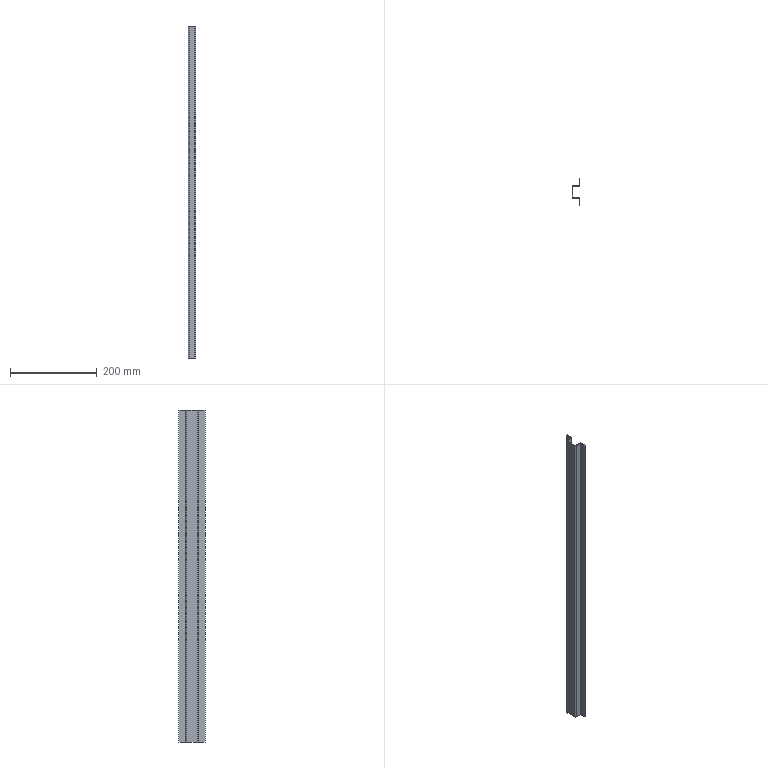Component | SolidWorks | UpperLeftSidePlate-1_UpperLeftOuterSidePanelStiffener-1 | 1 solid | 38 faces | box 18.4 x 60 x 766 mm | volume 104324 mm3 | plane 30 | cylinder 8 | commonest cylinder face diameters 5 x4 2 x4 | material 304
STEP:
#1=COLOUR_RGB('',0.7922,0.8196,0.9333);
#2=FILL_AREA_STYLE_COLOUR('',#1);
#3=FILL_AREA_STYLE('',(#2));
#4=SURFACE_STYLE_FILL_AREA(#3);
#5=SURFACE_SIDE_STYLE('',(#4));
#6=SURFACE_STYLE_USAGE(.BOTH.,#5);
#7=PRESENTATION_STYLE_ASSIGNMENT((#6));
#8=CARTESIAN_POINT('',(21.127,-3.735,78.388));
#9=VERTEX_POINT('',#8);
#10=CARTESIAN_POINT('',(21.127,-3.676,78.388));
#11=VERTEX_POINT('',#10);
#12=CARTESIAN_POINT('',(21.127,-3.735,78.388));
#13=DIRECTION('',(0.,1.,0.));
#14=VECTOR('',#13,39.37);
#15=LINE('',#12,#14);
#16=EDGE_CURVE('',#9,#11,#15,.T.);
#17=ORIENTED_EDGE('',*,*,#16,.F.);
#18=CARTESIAN_POINT('',(21.167,-3.775,78.388));
#19=VERTEX_POINT('',#18);
#20=CARTESIAN_POINT('',(21.127,-3.775,78.388));
#21=DIRECTION('',(-0.,0.,-1.));
#22=DIRECTION('',(-1.,0.,0.));
#23=AXIS2_PLACEMENT_3D('',#20,#21,#22);
#24=CIRCLE('',#23,0.03937);
#25=EDGE_CURVE('',#9,#19,#24,.T.);
#26=ORIENTED_EDGE('',*,*,#25,.T.);
#27=CARTESIAN_POINT('',(21.226,-3.775,78.388));
#28=VERTEX_POINT('',#27);
#29=CARTESIAN_POINT('',(21.226,-3.775,78.388));
#30=DIRECTION('',(-1.,0.,0.));
#31=VECTOR('',#30,39.37);
#32=LINE('',#29,#31);
#33=EDGE_CURVE('',#28,#19,#32,.T.);
#34=ORIENTED_EDGE('',*,*,#33,.F.);
#35=CARTESIAN_POINT('',(21.127,-3.775,78.388));
#36=DIRECTION('',(-0.,0.,-1.));
#37=DIRECTION('',(0.,1.,0.));
#38=AXIS2_PLACEMENT_3D('',#35,#36,#37);
#39=CIRCLE('',#38,0.09843);
#40=EDGE_CURVE('',#11,#28,#39,.T.);
#41=ORIENTED_EDGE('',*,*,#40,.F.);
#42=EDGE_LOOP('',(#17,#26,#34,#41));
#43=FACE_OUTER_BOUND('',#42,.T.);
#44=CARTESIAN_POINT('',(21.127,-3.735,78.388));
#45=DIRECTION('',(0.,-0.,1.));
#46=DIRECTION('',(1.,-0.,-0.));
#47=AXIS2_PLACEMENT_3D('',#44,#45,#46);
#48=PLANE('',#47);
#49=ADVANCED_FACE('',(#43),#48,.T.);
#50=CARTESIAN_POINT('',(20.6,-3.735,78.388));
#51=VERTEX_POINT('',#50);
#52=CARTESIAN_POINT('',(21.167,-3.735,78.388));
#53=DIRECTION('',(1.,-0.,-0.));
#54=VECTOR('',#53,39.37);
#55=LINE('',#52,#54);
#56=EDGE_CURVE('',#51,#9,#55,.T.);
#57=ORIENTED_EDGE('',*,*,#56,.T.);
#58=ORIENTED_EDGE('',*,*,#16,.T.);
#59=CARTESIAN_POINT('',(20.6,-3.676,78.388));
#60=VERTEX_POINT('',#59);
#61=CARTESIAN_POINT('',(21.167,-3.676,78.388));
#62=DIRECTION('',(1.,-0.,-0.));
#63=VECTOR('',#62,39.37);
#64=LINE('',#61,#63);
#65=EDGE_CURVE('',#60,#11,#64,.T.);
#66=ORIENTED_EDGE('',*,*,#65,.F.);
#67=CARTESIAN_POINT('',(20.6,-3.676,78.388));
#68=DIRECTION('',(-0.,-1.,-0.));
#69=VECTOR('',#68,39.37);
#70=LINE('',#67,#69);
#71=EDGE_CURVE('',#60,#51,#70,.T.);
#72=ORIENTED_EDGE('',*,*,#71,.T.);
#73=EDGE_LOOP('',(#57,#58,#66,#72));
#74=FACE_OUTER_BOUND('',#73,.T.);
#75=CARTESIAN_POINT('',(21.226,-3.775,78.388));
#76=DIRECTION('',(0.,-0.,1.));
#77=DIRECTION('',(1.,-0.,-0.));
#78=AXIS2_PLACEMENT_3D('',#75,#76,#77);
#79=PLANE('',#78);
#80=ADVANCED_FACE('',(#74),#79,.T.);
#81=CARTESIAN_POINT('',(21.167,-3.775,48.23));
#82=VERTEX_POINT('',#81);
#83=CARTESIAN_POINT('',(21.226,-3.775,48.23));
#84=VERTEX_POINT('',#83);
#85=CARTESIAN_POINT('',(21.167,-3.775,48.23));
#86=DIRECTION('',(1.,-0.,-0.));
#87=VECTOR('',#86,39.37);
#88=LINE('',#85,#87);
#89=EDGE_CURVE('',#82,#84,#88,.T.);
#90=ORIENTED_EDGE('',*,*,#89,.F.);
#91=CARTESIAN_POINT('',(21.127,-3.735,48.23));
#92=VERTEX_POINT('',#91);
#93=CARTESIAN_POINT('',(21.127,-3.775,48.23));
#94=DIRECTION('',(-0.,0.,-1.));
#95=DIRECTION('',(-1.,0.,0.));
#96=AXIS2_PLACEMENT_3D('',#93,#94,#95);
#97=CIRCLE('',#96,0.03937);
#98=EDGE_CURVE('',#92,#82,#97,.T.);
#99=ORIENTED_EDGE('',*,*,#98,.F.);
#100=CARTESIAN_POINT('',(21.127,-3.676,48.23));
#101=VERTEX_POINT('',#100);
#102=CARTESIAN_POINT('',(21.127,-3.676,48.23));
#103=DIRECTION('',(-0.,-1.,-0.));
#104=VECTOR('',#103,39.37);
#105=LINE('',#102,#104);
#106=EDGE_CURVE('',#101,#92,#105,.T.);
#107=ORIENTED_EDGE('',*,*,#106,.F.);
#108=CARTESIAN_POINT('',(21.127,-3.775,48.23));
#109=DIRECTION('',(-0.,0.,-1.));
#110=DIRECTION('',(0.,1.,0.));
#111=AXIS2_PLACEMENT_3D('',#108,#109,#110);
#112=CIRCLE('',#111,0.09843);
#113=EDGE_CURVE('',#101,#84,#112,.T.);
#114=ORIENTED_EDGE('',*,*,#113,.T.);
#115=EDGE_LOOP('',(#90,#99,#107,#114));
#116=FACE_OUTER_BOUND('',#115,.T.);
#117=CARTESIAN_POINT('',(21.167,-3.775,48.23));
#118=DIRECTION('',(-0.,0.,-1.));
#119=DIRECTION('',(-1.,0.,0.));
#120=AXIS2_PLACEMENT_3D('',#117,#118,#119);
#121=PLANE('',#120);
#122=ADVANCED_FACE('',(#116),#121,.T.);
#123=CARTESIAN_POINT('',(21.167,-4.326,48.23));
#124=VERTEX_POINT('',#123);
#125=CARTESIAN_POINT('',(21.167,-4.326,48.23));
#126=DIRECTION('',(-0.,-1.,-0.));
#127=VECTOR('',#126,39.37);
#128=LINE('',#125,#127);
#129=EDGE_CURVE('',#82,#124,#128,.T.);
#130=ORIENTED_EDGE('',*,*,#129,.F.);
#131=ORIENTED_EDGE('',*,*,#89,.T.);
#132=CARTESIAN_POINT('',(21.226,-4.326,48.23));
#133=VERTEX_POINT('',#132);
#134=CARTESIAN_POINT('',(21.226,-4.326,48.23));
#135=DIRECTION('',(-0.,-1.,-0.));
#136=VECTOR('',#135,39.37);
#137=LINE('',#134,#136);
#138=EDGE_CURVE('',#84,#133,#137,.T.);
#139=ORIENTED_EDGE('',*,*,#138,.T.);
#140=CARTESIAN_POINT('',(21.226,-4.326,48.23));
#141=DIRECTION('',(-1.,0.,0.));
#142=VECTOR('',#141,39.37);
#143=LINE('',#140,#142);
#144=EDGE_CURVE('',#133,#124,#143,.T.);
#145=ORIENTED_EDGE('',*,*,#144,.T.);
#146=EDGE_LOOP('',(#130,#131,#139,#145));
#147=FACE_OUTER_BOUND('',#146,.T.);
#148=CARTESIAN_POINT('',(21.127,-3.676,48.23));
#149=DIRECTION('',(-0.,0.,-1.));
#150=DIRECTION('',(-1.,0.,0.));
#151=AXIS2_PLACEMENT_3D('',#148,#149,#150);
#152=PLANE('',#151);
#153=ADVANCED_FACE('',(#147),#152,.T.);
#154=CARTESIAN_POINT('',(20.501,-3.637,78.388));
#155=VERTEX_POINT('',#154);
#156=CARTESIAN_POINT('',(20.56,-3.637,78.388));
#157=VERTEX_POINT('',#156);
#158=CARTESIAN_POINT('',(20.501,-3.637,78.388));
#159=DIRECTION('',(1.,-0.,-0.));
#160=VECTOR('',#159,39.37);
#161=LINE('',#158,#160);
#162=EDGE_CURVE('',#155,#157,#161,.T.);
#163=ORIENTED_EDGE('',*,*,#162,.F.);
#164=CARTESIAN_POINT('',(20.6,-3.637,78.388));
#165=DIRECTION('',(0.,-0.,1.));
#166=DIRECTION('',(1.,-0.,0.));
#167=AXIS2_PLACEMENT_3D('',#164,#165,#166);
#168=CIRCLE('',#167,0.09843);
#169=EDGE_CURVE('',#155,#51,#168,.T.);
#170=ORIENTED_EDGE('',*,*,#169,.T.);
#171=ORIENTED_EDGE('',*,*,#71,.F.);
#172=CARTESIAN_POINT('',(20.6,-3.637,78.388));
#173=DIRECTION('',(0.,-0.,1.));
#174=DIRECTION('',(0.,1.,0.));
#175=AXIS2_PLACEMENT_3D('',#172,#173,#174);
#176=CIRCLE('',#175,0.03937);
#177=EDGE_CURVE('',#157,#60,#176,.T.);
#178=ORIENTED_EDGE('',*,*,#177,.F.);
#179=EDGE_LOOP('',(#163,#170,#171,#178));
#180=FACE_OUTER_BOUND('',#179,.T.);
#181=CARTESIAN_POINT('',(20.501,-3.637,78.388));
#182=DIRECTION('',(0.,-0.,1.));
#183=DIRECTION('',(1.,-0.,-0.));
#184=AXIS2_PLACEMENT_3D('',#181,#182,#183);
#185=PLANE('',#184);
#186=ADVANCED_FACE('',(#180),#185,.T.);
#187=CARTESIAN_POINT('',(20.501,-2.653,78.388));
#188=VERTEX_POINT('',#187);
#189=CARTESIAN_POINT('',(20.501,-3.735,78.388));
#190=DIRECTION('',(-0.,-1.,-0.));
#191=VECTOR('',#190,39.37);
#192=LINE('',#189,#191);
#193=EDGE_CURVE('',#188,#155,#192,.T.);
#194=ORIENTED_EDGE('',*,*,#193,.T.);
#195=ORIENTED_EDGE('',*,*,#162,.T.);
#196=CARTESIAN_POINT('',(20.56,-2.653,78.388));
#197=VERTEX_POINT('',#196);
#198=CARTESIAN_POINT('',(20.56,-3.735,78.388));
#199=DIRECTION('',(-0.,-1.,-0.));
#200=VECTOR('',#199,39.37);
#201=LINE('',#198,#200);
#202=EDGE_CURVE('',#197,#157,#201,.T.);
#203=ORIENTED_EDGE('',*,*,#202,.F.);
#204=CARTESIAN_POINT('',(20.56,-2.653,78.388));
#205=DIRECTION('',(-1.,0.,0.));
#206=VECTOR('',#205,39.37);
#207=LINE('',#204,#206);
#208=EDGE_CURVE('',#197,#188,#207,.T.);
#209=ORIENTED_EDGE('',*,*,#208,.T.);
#210=EDGE_LOOP('',(#194,#195,#203,#209));
#211=FACE_OUTER_BOUND('',#210,.T.);
#212=CARTESIAN_POINT('',(20.6,-3.676,78.388));
#213=DIRECTION('',(0.,-0.,1.));
#214=DIRECTION('',(1.,-0.,-0.));
#215=AXIS2_PLACEMENT_3D('',#212,#213,#214);
#216=PLANE('',#215);
#217=ADVANCED_FACE('',(#211),#216,.T.);
#218=CARTESIAN_POINT('',(20.6,-3.735,48.23));
#219=VERTEX_POINT('',#218);
#220=CARTESIAN_POINT('',(20.6,-3.676,48.23));
#221=VERTEX_POINT('',#220);
#222=CARTESIAN_POINT('',(20.6,-3.735,48.23));
#223=DIRECTION('',(0.,1.,0.));
#224=VECTOR('',#223,39.37);
#225=LINE('',#222,#224);
#226=EDGE_CURVE('',#219,#221,#225,.T.);
#227=ORIENTED_EDGE('',*,*,#226,.F.);
#228=CARTESIAN_POINT('',(20.501,-3.637,48.23));
#229=VERTEX_POINT('',#228);
#230=CARTESIAN_POINT('',(20.6,-3.637,48.23));
#231=DIRECTION('',(0.,-0.,1.));
#232=DIRECTION('',(1.,-0.,0.));
#233=AXIS2_PLACEMENT_3D('',#230,#231,#232);
#234=CIRCLE('',#233,0.09843);
#235=EDGE_CURVE('',#229,#219,#234,.T.);
#236=ORIENTED_EDGE('',*,*,#235,.F.);
#237=CARTESIAN_POINT('',(20.56,-3.637,48.23));
#238=VERTEX_POINT('',#237);
#239=CARTESIAN_POINT('',(20.56,-3.637,48.23));
#240=DIRECTION('',(-1.,0.,0.));
#241=VECTOR('',#240,39.37);
#242=LINE('',#239,#241);
#243=EDGE_CURVE('',#238,#229,#242,.T.);
#244=ORIENTED_EDGE('',*,*,#243,.F.);
#245=CARTESIAN_POINT('',(20.6,-3.637,48.23));
#246=DIRECTION('',(0.,-0.,1.));
#247=DIRECTION('',(0.,1.,0.));
#248=AXIS2_PLACEMENT_3D('',#245,#246,#247);
#249=CIRCLE('',#248,0.03937);
#250=EDGE_CURVE('',#238,#221,#249,.T.);
#251=ORIENTED_EDGE('',*,*,#250,.T.);
#252=EDGE_LOOP('',(#227,#236,#244,#251));
#253=FACE_OUTER_BOUND('',#252,.T.);
#254=CARTESIAN_POINT('',(20.6,-3.735,48.23));
#255=DIRECTION('',(-0.,0.,-1.));
#256=DIRECTION('',(-1.,0.,0.));
#257=AXIS2_PLACEMENT_3D('',#254,#255,#256);
#258=PLANE('',#257);
#259=ADVANCED_FACE('',(#253),#258,.T.);
#260=CARTESIAN_POINT('',(21.167,-3.735,48.23));
#261=DIRECTION('',(1.,-0.,-0.));
#262=VECTOR('',#261,39.37);
#263=LINE('',#260,#262);
#264=EDGE_CURVE('',#219,#92,#263,.T.);
#265=ORIENTED_EDGE('',*,*,#264,.F.);
#266=ORIENTED_EDGE('',*,*,#226,.T.);
#267=CARTESIAN_POINT('',(21.167,-3.676,48.23));
#268=DIRECTION('',(1.,-0.,-0.));
#269=VECTOR('',#268,39.37);
#270=LINE('',#267,#269);
#271=EDGE_CURVE('',#221,#101,#270,.T.);
#272=ORIENTED_EDGE('',*,*,#271,.T.);
#273=ORIENTED_EDGE('',*,*,#106,.T.);
#274=EDGE_LOOP('',(#265,#266,#272,#273));
#275=FACE_OUTER_BOUND('',#274,.T.);
#276=CARTESIAN_POINT('',(20.56,-3.637,48.23));
#277=DIRECTION('',(-0.,0.,-1.));
#278=DIRECTION('',(-1.,0.,0.));
#279=AXIS2_PLACEMENT_3D('',#276,#277,#278);
#280=PLANE('',#279);
#281=ADVANCED_FACE('',(#275),#280,.T.);
#282=CARTESIAN_POINT('',(20.6,-2.554,78.388));
#283=VERTEX_POINT('',#282);
#284=CARTESIAN_POINT('',(20.6,-2.613,78.388));
#285=VERTEX_POINT('',#284);
#286=CARTESIAN_POINT('',(20.6,-2.554,78.388));
#287=DIRECTION('',(-0.,-1.,-0.));
#288=VECTOR('',#287,39.37);
#289=LINE('',#286,#288);
#290=EDGE_CURVE('',#283,#285,#289,.T.);
#291=ORIENTED_EDGE('',*,*,#290,.F.);
#292=CARTESIAN_POINT('',(20.6,-2.653,78.388));
#293=DIRECTION('',(0.,-0.,1.));
#294=DIRECTION('',(1.,-0.,0.));
#295=AXIS2_PLACEMENT_3D('',#292,#293,#294);
#296=CIRCLE('',#295,0.09843);
#297=EDGE_CURVE('',#283,#188,#296,.T.);
#298=ORIENTED_EDGE('',*,*,#297,.T.);
#299=ORIENTED_EDGE('',*,*,#208,.F.);
#300=CARTESIAN_POINT('',(20.6,-2.653,78.388));
#301=DIRECTION('',(0.,-0.,1.));
#302=DIRECTION('',(0.,1.,0.));
#303=AXIS2_PLACEMENT_3D('',#300,#301,#302);
#304=CIRCLE('',#303,0.03937);
#305=EDGE_CURVE('',#285,#197,#304,.T.);
#306=ORIENTED_EDGE('',*,*,#305,.F.);
#307=EDGE_LOOP('',(#291,#298,#299,#306));
#308=FACE_OUTER_BOUND('',#307,.T.);
#309=CARTESIAN_POINT('',(20.6,-2.554,78.388));
#310=DIRECTION('',(0.,-0.,1.));
#311=DIRECTION('',(1.,-0.,-0.));
#312=AXIS2_PLACEMENT_3D('',#309,#310,#311);
#313=PLANE('',#312);
#314=ADVANCED_FACE('',(#308),#313,.T.);
#315=CARTESIAN_POINT('',(21.127,-2.554,78.388));
#316=VERTEX_POINT('',#315);
#317=CARTESIAN_POINT('',(21.167,-2.554,78.388));
#318=DIRECTION('',(-1.,0.,0.));
#319=VECTOR('',#318,39.37);
#320=LINE('',#317,#319);
#321=EDGE_CURVE('',#316,#283,#320,.T.);
#322=ORIENTED_EDGE('',*,*,#321,.T.);
#323=ORIENTED_EDGE('',*,*,#290,.T.);
#324=CARTESIAN_POINT('',(21.127,-2.613,78.388));
#325=VERTEX_POINT('',#324);
#326=CARTESIAN_POINT('',(21.167,-2.613,78.388));
#327=DIRECTION('',(-1.,0.,0.));
#328=VECTOR('',#327,39.37);
#329=LINE('',#326,#328);
#330=EDGE_CURVE('',#325,#285,#329,.T.);
#331=ORIENTED_EDGE('',*,*,#330,.F.);
#332=CARTESIAN_POINT('',(21.127,-2.613,78.388));
#333=DIRECTION('',(0.,1.,0.));
#334=VECTOR('',#333,39.37);
#335=LINE('',#332,#334);
#336=EDGE_CURVE('',#325,#316,#335,.T.);
#337=ORIENTED_EDGE('',*,*,#336,.T.);
#338=EDGE_LOOP('',(#322,#323,#331,#337));
#339=FACE_OUTER_BOUND('',#338,.T.);
#340=CARTESIAN_POINT('',(20.56,-2.653,78.388));
#341=DIRECTION('',(0.,-0.,1.));
#342=DIRECTION('',(1.,-0.,-0.));
#343=AXIS2_PLACEMENT_3D('',#340,#341,#342);
#344=PLANE('',#343);
#345=ADVANCED_FACE('',(#339),#344,.T.);
#346=CARTESIAN_POINT('',(20.501,-2.653,48.23));
#347=VERTEX_POINT('',#346);
#348=CARTESIAN_POINT('',(20.56,-2.653,48.23));
#349=VERTEX_POINT('',#348);
#350=CARTESIAN_POINT('',(20.501,-2.653,48.23));
#351=DIRECTION('',(1.,-0.,-0.));
#352=VECTOR('',#351,39.37);
#353=LINE('',#350,#352);
#354=EDGE_CURVE('',#347,#349,#353,.T.);
#355=ORIENTED_EDGE('',*,*,#354,.F.);
#356=CARTESIAN_POINT('',(20.6,-2.554,48.23));
#357=VERTEX_POINT('',#356);
#358=CARTESIAN_POINT('',(20.6,-2.653,48.23));
#359=DIRECTION('',(0.,-0.,1.));
#360=DIRECTION('',(1.,-0.,0.));
#361=AXIS2_PLACEMENT_3D('',#358,#359,#360);
#362=CIRCLE('',#361,0.09843);
#363=EDGE_CURVE('',#357,#347,#362,.T.);
#364=ORIENTED_EDGE('',*,*,#363,.F.);
#365=CARTESIAN_POINT('',(20.6,-2.613,48.23));
#366=VERTEX_POINT('',#365);
#367=CARTESIAN_POINT('',(20.6,-2.613,48.23));
#368=DIRECTION('',(0.,1.,0.));
#369=VECTOR('',#368,39.37);
#370=LINE('',#367,#369);
#371=EDGE_CURVE('',#366,#357,#370,.T.);
#372=ORIENTED_EDGE('',*,*,#371,.F.);
#373=CARTESIAN_POINT('',(20.6,-2.653,48.23));
#374=DIRECTION('',(0.,-0.,1.));
#375=DIRECTION('',(0.,1.,0.));
#376=AXIS2_PLACEMENT_3D('',#373,#374,#375);
#377=CIRCLE('',#376,0.03937);
#378=EDGE_CURVE('',#366,#349,#377,.T.);
#379=ORIENTED_EDGE('',*,*,#378,.T.);
#380=EDGE_LOOP('',(#355,#364,#372,#379));
#381=FACE_OUTER_BOUND('',#380,.T.);
#382=CARTESIAN_POINT('',(20.501,-2.653,48.23));
#383=DIRECTION('',(-0.,0.,-1.));
#384=DIRECTION('',(-1.,0.,0.));
#385=AXIS2_PLACEMENT_3D('',#382,#383,#384);
#386=PLANE('',#385);
#387=ADVANCED_FACE('',(#381),#386,.T.);
#388=CARTESIAN_POINT('',(20.501,-3.735,48.23));
#389=DIRECTION('',(-0.,-1.,-0.));
#390=VECTOR('',#389,39.37);
#391=LINE('',#388,#390);
#392=EDGE_CURVE('',#347,#229,#391,.T.);
#393=ORIENTED_EDGE('',*,*,#392,.F.);
#394=ORIENTED_EDGE('',*,*,#354,.T.);
#395=CARTESIAN_POINT('',(20.56,-3.735,48.23));
#396=DIRECTION('',(-0.,-1.,-0.));
#397=VECTOR('',#396,39.37);
#398=LINE('',#395,#397);
#399=EDGE_CURVE('',#349,#238,#398,.T.);
#400=ORIENTED_EDGE('',*,*,#399,.T.);
#401=ORIENTED_EDGE('',*,*,#243,.T.);
#402=EDGE_LOOP('',(#393,#394,#400,#401));
#403=FACE_OUTER_BOUND('',#402,.T.);
#404=CARTESIAN_POINT('',(20.6,-2.613,48.23));
#405=DIRECTION('',(-0.,0.,-1.));
#406=DIRECTION('',(-1.,0.,0.));
#407=AXIS2_PLACEMENT_3D('',#404,#405,#406);
#408=PLANE('',#407);
#409=ADVANCED_FACE('',(#403),#408,.T.);
#410=CARTESIAN_POINT('',(21.167,-2.515,78.388));
#411=VERTEX_POINT('',#410);
#412=CARTESIAN_POINT('',(21.226,-2.515,78.388));
#413=VERTEX_POINT('',#412);
#414=CARTESIAN_POINT('',(21.167,-2.515,78.388));
#415=DIRECTION('',(1.,0.,-0.));
#416=VECTOR('',#415,39.37);
#417=LINE('',#414,#416);
#418=EDGE_CURVE('',#411,#413,#417,.T.);
#419=ORIENTED_EDGE('',*,*,#418,.F.);
#420=CARTESIAN_POINT('',(21.127,-2.515,78.388));
#421=DIRECTION('',(-0.,0.,-1.));
#422=DIRECTION('',(-1.,0.,0.));
#423=AXIS2_PLACEMENT_3D('',#420,#421,#422);
#424=CIRCLE('',#423,0.03937);
#425=EDGE_CURVE('',#411,#316,#424,.T.);
#426=ORIENTED_EDGE('',*,*,#425,.T.);
#427=ORIENTED_EDGE('',*,*,#336,.F.);
#428=CARTESIAN_POINT('',(21.127,-2.515,78.388));
#429=DIRECTION('',(-0.,0.,-1.));
#430=DIRECTION('',(0.,1.,0.));
#431=AXIS2_PLACEMENT_3D('',#428,#429,#430);
#432=CIRCLE('',#431,0.09843);
#433=EDGE_CURVE('',#413,#325,#432,.T.);
#434=ORIENTED_EDGE('',*,*,#433,.F.);
#435=EDGE_LOOP('',(#419,#426,#427,#434));
#436=FACE_OUTER_BOUND('',#435,.T.);
#437=CARTESIAN_POINT('',(21.167,-2.515,78.388));
#438=DIRECTION('',(0.,-0.,1.));
#439=DIRECTION('',(1.,-0.,-0.));
#440=AXIS2_PLACEMENT_3D('',#437,#438,#439);
#441=PLANE('',#440);
#442=ADVANCED_FACE('',(#436),#441,.T.);
#443=CARTESIAN_POINT('',(21.167,-1.964,78.388));
#444=VERTEX_POINT('',#443);
#445=CARTESIAN_POINT('',(21.167,-1.964,78.388));
#446=DIRECTION('',(-0.,-1.,-0.));
#447=VECTOR('',#446,39.37);
#448=LINE('',#445,#447);
#449=EDGE_CURVE('',#444,#411,#448,.T.);
#450=ORIENTED_EDGE('',*,*,#449,.T.);
#451=ORIENTED_EDGE('',*,*,#418,.T.);
#452=CARTESIAN_POINT('',(21.226,-1.964,78.388));
#453=VERTEX_POINT('',#452);
#454=CARTESIAN_POINT('',(21.226,-1.964,78.388));
#455=DIRECTION('',(-0.,-1.,-0.));
#456=VECTOR('',#455,39.37);
#457=LINE('',#454,#456);
#458=EDGE_CURVE('',#453,#413,#457,.T.);
#459=ORIENTED_EDGE('',*,*,#458,.F.);
#460=CARTESIAN_POINT('',(21.167,-1.964,78.388));
#461=DIRECTION('',(1.,-0.,-0.));
#462=VECTOR('',#461,39.37);
#463=LINE('',#460,#462);
#464=EDGE_CURVE('',#444,#453,#463,.T.);
#465=ORIENTED_EDGE('',*,*,#464,.F.);
#466=EDGE_LOOP('',(#450,#451,#459,#465));
#467=FACE_OUTER_BOUND('',#466,.T.);
#468=CARTESIAN_POINT('',(21.127,-2.613,78.388));
#469=DIRECTION('',(0.,-0.,1.));
#470=DIRECTION('',(1.,-0.,-0.));
#471=AXIS2_PLACEMENT_3D('',#468,#469,#470);
#472=PLANE('',#471);
#473=ADVANCED_FACE('',(#467),#472,.T.);
#474=CARTESIAN_POINT('',(21.127,-2.554,48.23));
#475=VERTEX_POINT('',#474);
#476=CARTESIAN_POINT('',(21.127,-2.613,48.23));
#477=VERTEX_POINT('',#476);
#478=CARTESIAN_POINT('',(21.127,-2.554,48.23));
#479=DIRECTION('',(-0.,-1.,-0.));
#480=VECTOR('',#479,39.37);
#481=LINE('',#478,#480);
#482=EDGE_CURVE('',#475,#477,#481,.T.);
#483=ORIENTED_EDGE('',*,*,#482,.F.);
#484=CARTESIAN_POINT('',(21.167,-2.515,48.23));
#485=VERTEX_POINT('',#484);
#486=CARTESIAN_POINT('',(21.127,-2.515,48.23));
#487=DIRECTION('',(-0.,0.,-1.));
#488=DIRECTION('',(-1.,0.,0.));
#489=AXIS2_PLACEMENT_3D('',#486,#487,#488);
#490=CIRCLE('',#489,0.03937);
#491=EDGE_CURVE('',#485,#475,#490,.T.);
#492=ORIENTED_EDGE('',*,*,#491,.F.);
#493=CARTESIAN_POINT('',(21.226,-2.515,48.23));
#494=VERTEX_POINT('',#493);
#495=CARTESIAN_POINT('',(21.226,-2.515,48.23));
#496=DIRECTION('',(-1.,-0.,0.));
#497=VECTOR('',#496,39.37);
#498=LINE('',#495,#497);
#499=EDGE_CURVE('',#494,#485,#498,.T.);
#500=ORIENTED_EDGE('',*,*,#499,.F.);
#501=CARTESIAN_POINT('',(21.127,-2.515,48.23));
#502=DIRECTION('',(-0.,0.,-1.));
#503=DIRECTION('',(0.,1.,0.));
#504=AXIS2_PLACEMENT_3D('',#501,#502,#503);
#505=CIRCLE('',#504,0.09843);
#506=EDGE_CURVE('',#494,#477,#505,.T.);
#507=ORIENTED_EDGE('',*,*,#506,.T.);
#508=EDGE_LOOP('',(#483,#492,#500,#507));
#509=FACE_OUTER_BOUND('',#508,.T.);
#510=CARTESIAN_POINT('',(21.127,-2.554,48.23));
#511=DIRECTION('',(-0.,0.,-1.));
#512=DIRECTION('',(-1.,0.,0.));
#513=AXIS2_PLACEMENT_3D('',#510,#511,#512);
#514=PLANE('',#513);
#515=ADVANCED_FACE('',(#509),#514,.T.);
#516=CARTESIAN_POINT('',(21.167,-2.554,48.23));
#517=DIRECTION('',(-1.,0.,0.));
#518=VECTOR('',#517,39.37);
#519=LINE('',#516,#518);
#520=EDGE_CURVE('',#475,#357,#519,.T.);
#521=ORIENTED_EDGE('',*,*,#520,.F.);
#522=ORIENTED_EDGE('',*,*,#482,.T.);
#523=CARTESIAN_POINT('',(21.167,-2.613,48.23));
#524=DIRECTION('',(-1.,0.,0.));
#525=VECTOR('',#524,39.37);
#526=LINE('',#523,#525);
#527=EDGE_CURVE('',#477,#366,#526,.T.);
#528=ORIENTED_EDGE('',*,*,#527,.T.);
#529=ORIENTED_EDGE('',*,*,#371,.T.);
#530=EDGE_LOOP('',(#521,#522,#528,#529));
#531=FACE_OUTER_BOUND('',#530,.T.);
#532=CARTESIAN_POINT('',(21.226,-2.515,48.23));
#533=DIRECTION('',(-0.,0.,-1.));
#534=DIRECTION('',(-1.,0.,0.));
#535=AXIS2_PLACEMENT_3D('',#532,#533,#534);
#536=PLANE('',#535);
#537=ADVANCED_FACE('',(#531),#536,.T.);
#538=ORIENTED_EDGE('',*,*,#129,.T.);
#539=CARTESIAN_POINT('',(21.167,-4.326,78.388));
#540=VERTEX_POINT('',#539);
#541=CARTESIAN_POINT('',(21.167,-4.326,78.388));
#542=DIRECTION('',(-0.,0.,-1.));
#543=VECTOR('',#542,39.37);
#544=LINE('',#541,#543);
#545=EDGE_CURVE('',#540,#124,#544,.T.);
#546=ORIENTED_EDGE('',*,*,#545,.F.);
#547=CARTESIAN_POINT('',(21.167,-4.326,78.388));
#548=DIRECTION('',(-0.,-1.,-0.));
#549=VECTOR('',#548,39.37);
#550=LINE('',#547,#549);
#551=EDGE_CURVE('',#19,#540,#550,.T.);
#552=ORIENTED_EDGE('',*,*,#551,.F.);
#553=CARTESIAN_POINT('',(21.167,-3.775,78.388));
#554=DIRECTION('',(-0.,0.,-1.));
#555=VECTOR('',#554,39.37);
#556=LINE('',#553,#555);
#557=EDGE_CURVE('',#19,#82,#556,.T.);
#558=ORIENTED_EDGE('',*,*,#557,.T.);
#559=EDGE_LOOP('',(#538,#546,#552,#558));
#560=FACE_OUTER_BOUND('',#559,.T.);
#561=CARTESIAN_POINT('',(21.167,-4.326,78.388));
#562=DIRECTION('',(1.,-0.,-0.));
#563=DIRECTION('',(0.,1.,0.));
#564=AXIS2_PLACEMENT_3D('',#561,#562,#563);
#565=PLANE('',#564);
#566=ADVANCED_FACE('',(#560),#565,.F.);
#567=ORIENTED_EDGE('',*,*,#144,.F.);
#568=CARTESIAN_POINT('',(21.226,-4.326,78.388));
#569=VERTEX_POINT('',#568);
#570=CARTESIAN_POINT('',(21.226,-4.326,78.388));
#571=DIRECTION('',(-0.,0.,-1.));
#572=VECTOR('',#571,39.37);
#573=LINE('',#570,#572);
#574=EDGE_CURVE('',#569,#133,#573,.T.);
#575=ORIENTED_EDGE('',*,*,#574,.F.);
#576=CARTESIAN_POINT('',(21.226,-4.326,78.388));
#577=DIRECTION('',(-1.,0.,0.));
#578=VECTOR('',#577,39.37);
#579=LINE('',#576,#578);
#580=EDGE_CURVE('',#569,#540,#579,.T.);
#581=ORIENTED_EDGE('',*,*,#580,.T.);
#582=ORIENTED_EDGE('',*,*,#545,.T.);
#583=EDGE_LOOP('',(#567,#575,#581,#582));
#584=FACE_OUTER_BOUND('',#583,.T.);
#585=CARTESIAN_POINT('',(21.226,-4.326,78.388));
#586=DIRECTION('',(-0.,-1.,-0.));
#587=DIRECTION('',(1.,-0.,-0.));
#588=AXIS2_PLACEMENT_3D('',#585,#586,#587);
#589=PLANE('',#588);
#590=ADVANCED_FACE('',(#584),#589,.T.);
#591=ORIENTED_EDGE('',*,*,#138,.F.);
#592=CARTESIAN_POINT('',(21.226,-3.775,78.388));
#593=DIRECTION('',(-0.,0.,-1.));
#594=VECTOR('',#593,39.37);
#595=LINE('',#592,#594);
#596=EDGE_CURVE('',#28,#84,#595,.T.);
#597=ORIENTED_EDGE('',*,*,#596,.F.);
#598=CARTESIAN_POINT('',(21.226,-4.326,78.388));
#599=DIRECTION('',(-0.,-1.,-0.));
#600=VECTOR('',#599,39.37);
#601=LINE('',#598,#600);
#602=EDGE_CURVE('',#28,#569,#601,.T.);
#603=ORIENTED_EDGE('',*,*,#602,.T.);
#604=ORIENTED_EDGE('',*,*,#574,.T.);
#605=EDGE_LOOP('',(#591,#597,#603,#604));
#606=FACE_OUTER_BOUND('',#605,.T.);
#607=CARTESIAN_POINT('',(21.226,-4.326,78.388));
#608=DIRECTION('',(1.,-0.,-0.));
#609=DIRECTION('',(0.,1.,0.));
#610=AXIS2_PLACEMENT_3D('',#607,#608,#609);
#611=PLANE('',#610);
#612=ADVANCED_FACE('',(#606),#611,.T.);
#613=ORIENTED_EDGE('',*,*,#113,.F.);
#614=CARTESIAN_POINT('',(21.127,-3.676,78.388));
#615=DIRECTION('',(-0.,0.,-1.));
#616=VECTOR('',#615,39.37);
#617=LINE('',#614,#616);
#618=EDGE_CURVE('',#11,#101,#617,.T.);
#619=ORIENTED_EDGE('',*,*,#618,.F.);
#620=ORIENTED_EDGE('',*,*,#40,.T.);
#621=ORIENTED_EDGE('',*,*,#596,.T.);
#622=EDGE_LOOP('',(#613,#619,#620,#621));
#623=FACE_OUTER_BOUND('',#622,.T.);
#624=CARTESIAN_POINT('',(21.127,-3.775,78.388));
#625=DIRECTION('',(-0.,0.,-1.));
#626=DIRECTION('',(-1.,0.,0.));
#627=AXIS2_PLACEMENT_3D('',#624,#625,#626);
#628=CYLINDRICAL_SURFACE('',#627,0.09843);
#629=ADVANCED_FACE('',(#623),#628,.T.);
#630=ORIENTED_EDGE('',*,*,#271,.F.);
#631=CARTESIAN_POINT('',(20.6,-3.676,78.388));
#632=DIRECTION('',(-0.,0.,-1.));
#633=VECTOR('',#632,39.37);
#634=LINE('',#631,#633);
#635=EDGE_CURVE('',#60,#221,#634,.T.);
#636=ORIENTED_EDGE('',*,*,#635,.F.);
#637=ORIENTED_EDGE('',*,*,#65,.T.);
#638=ORIENTED_EDGE('',*,*,#618,.T.);
#639=EDGE_LOOP('',(#630,#636,#637,#638));
#640=FACE_OUTER_BOUND('',#639,.T.);
#641=CARTESIAN_POINT('',(21.167,-3.676,78.388));
#642=DIRECTION('',(0.,1.,0.));
#643=DIRECTION('',(-1.,0.,0.));
#644=AXIS2_PLACEMENT_3D('',#641,#642,#643);
#645=PLANE('',#644);
#646=ADVANCED_FACE('',(#640),#645,.T.);
#647=ORIENTED_EDGE('',*,*,#250,.F.);
#648=CARTESIAN_POINT('',(20.56,-3.637,78.388));
#649=DIRECTION('',(-0.,0.,-1.));
#650=VECTOR('',#649,39.37);
#651=LINE('',#648,#650);
#652=EDGE_CURVE('',#157,#238,#651,.T.);
#653=ORIENTED_EDGE('',*,*,#652,.F.);
#654=ORIENTED_EDGE('',*,*,#177,.T.);
#655=ORIENTED_EDGE('',*,*,#635,.T.);
#656=EDGE_LOOP('',(#647,#653,#654,#655));
#657=FACE_OUTER_BOUND('',#656,.T.);
#658=CARTESIAN_POINT('',(20.6,-3.637,78.388));
#659=DIRECTION('',(-0.,0.,-1.));
#660=DIRECTION('',(-1.,0.,0.));
#661=AXIS2_PLACEMENT_3D('',#658,#659,#660);
#662=CYLINDRICAL_SURFACE('',#661,0.03937);
#663=ADVANCED_FACE('',(#657),#662,.F.);
#664=ORIENTED_EDGE('',*,*,#399,.F.);
#665=CARTESIAN_POINT('',(20.56,-2.653,78.388));
#666=DIRECTION('',(-0.,0.,-1.));
#667=VECTOR('',#666,39.37);
#668=LINE('',#665,#667);
#669=EDGE_CURVE('',#197,#349,#668,.T.);
#670=ORIENTED_EDGE('',*,*,#669,.F.);
#671=ORIENTED_EDGE('',*,*,#202,.T.);
#672=ORIENTED_EDGE('',*,*,#652,.T.);
#673=EDGE_LOOP('',(#664,#670,#671,#672));
#674=FACE_OUTER_BOUND('',#673,.T.);
#675=CARTESIAN_POINT('',(20.56,-3.735,78.388));
#676=DIRECTION('',(1.,-0.,-0.));
#677=DIRECTION('',(0.,1.,0.));
#678=AXIS2_PLACEMENT_3D('',#675,#676,#677);
#679=PLANE('',#678);
#680=ADVANCED_FACE('',(#674),#679,.T.);
#681=ORIENTED_EDGE('',*,*,#378,.F.);
#682=CARTESIAN_POINT('',(20.6,-2.613,78.388));
#683=DIRECTION('',(-0.,0.,-1.));
#684=VECTOR('',#683,39.37);
#685=LINE('',#682,#684);
#686=EDGE_CURVE('',#285,#366,#685,.T.);
#687=ORIENTED_EDGE('',*,*,#686,.F.);
#688=ORIENTED_EDGE('',*,*,#305,.T.);
#689=ORIENTED_EDGE('',*,*,#669,.T.);
#690=EDGE_LOOP('',(#681,#687,#688,#689));
#691=FACE_OUTER_BOUND('',#690,.T.);
#692=CARTESIAN_POINT('',(20.6,-2.653,78.388));
#693=DIRECTION('',(-0.,0.,-1.));
#694=DIRECTION('',(-1.,0.,0.));
#695=AXIS2_PLACEMENT_3D('',#692,#693,#694);
#696=CYLINDRICAL_SURFACE('',#695,0.03937);
#697=ADVANCED_FACE('',(#691),#696,.F.);
#698=ORIENTED_EDGE('',*,*,#527,.F.);
#699=CARTESIAN_POINT('',(21.127,-2.613,78.388));
#700=DIRECTION('',(-0.,0.,-1.));
#701=VECTOR('',#700,39.37);
#702=LINE('',#699,#701);
#703=EDGE_CURVE('',#325,#477,#702,.T.);
#704=ORIENTED_EDGE('',*,*,#703,.F.);
#705=ORIENTED_EDGE('',*,*,#330,.T.);
#706=ORIENTED_EDGE('',*,*,#686,.T.);
#707=EDGE_LOOP('',(#698,#704,#705,#706));
#708=FACE_OUTER_BOUND('',#707,.T.);
#709=CARTESIAN_POINT('',(21.167,-2.613,78.388));
#710=DIRECTION('',(-0.,-1.,-0.));
#711=DIRECTION('',(1.,-0.,-0.));
#712=AXIS2_PLACEMENT_3D('',#709,#710,#711);
#713=PLANE('',#712);
#714=ADVANCED_FACE('',(#708),#713,.T.);
#715=ORIENTED_EDGE('',*,*,#506,.F.);
#716=CARTESIAN_POINT('',(21.226,-2.515,78.388));
#717=DIRECTION('',(-0.,0.,-1.));
#718=VECTOR('',#717,39.37);
#719=LINE('',#716,#718);
#720=EDGE_CURVE('',#413,#494,#719,.T.);
#721=ORIENTED_EDGE('',*,*,#720,.F.);
#722=ORIENTED_EDGE('',*,*,#433,.T.);
#723=ORIENTED_EDGE('',*,*,#703,.T.);
#724=EDGE_LOOP('',(#715,#721,#722,#723));
#725=FACE_OUTER_BOUND('',#724,.T.);
#726=CARTESIAN_POINT('',(21.127,-2.515,78.388));
#727=DIRECTION('',(-0.,0.,-1.));
#728=DIRECTION('',(-1.,0.,0.));
#729=AXIS2_PLACEMENT_3D('',#726,#727,#728);
#730=CYLINDRICAL_SURFACE('',#729,0.09843);
#731=ADVANCED_FACE('',(#725),#730,.T.);
#732=CARTESIAN_POINT('',(21.226,-1.964,48.23));
#733=VERTEX_POINT('',#732);
#734=CARTESIAN_POINT('',(21.226,-1.964,48.23));
#735=DIRECTION('',(-0.,-1.,-0.));
#736=VECTOR('',#735,39.37);
#737=LINE('',#734,#736);
#738=EDGE_CURVE('',#733,#494,#737,.T.);
#739=ORIENTED_EDGE('',*,*,#738,.F.);
#740=CARTESIAN_POINT('',(21.226,-1.964,78.388));
#741=DIRECTION('',(-0.,0.,-1.));
#742=VECTOR('',#741,39.37);
#743=LINE('',#740,#742);
#744=EDGE_CURVE('',#453,#733,#743,.T.);
#745=ORIENTED_EDGE('',*,*,#744,.F.);
#746=ORIENTED_EDGE('',*,*,#458,.T.);
#747=ORIENTED_EDGE('',*,*,#720,.T.);
#748=EDGE_LOOP('',(#739,#745,#746,#747));
#749=FACE_OUTER_BOUND('',#748,.T.);
#750=CARTESIAN_POINT('',(21.226,-1.964,78.388));
#751=DIRECTION('',(1.,-0.,-0.));
#752=DIRECTION('',(0.,1.,0.));
#753=AXIS2_PLACEMENT_3D('',#750,#751,#752);
#754=PLANE('',#753);
#755=ADVANCED_FACE('',(#749),#754,.T.);
#756=CARTESIAN_POINT('',(21.167,-1.964,48.23));
#757=VERTEX_POINT('',#756);
#758=CARTESIAN_POINT('',(21.167,-1.964,48.23));
#759=DIRECTION('',(1.,-0.,-0.));
#760=VECTOR('',#759,39.37);
#761=LINE('',#758,#760);
#762=EDGE_CURVE('',#757,#733,#761,.T.);
#763=ORIENTED_EDGE('',*,*,#762,.F.);
#764=CARTESIAN_POINT('',(21.167,-1.964,78.388));
#765=DIRECTION('',(-0.,0.,-1.));
#766=VECTOR('',#765,39.37);
#767=LINE('',#764,#766);
#768=EDGE_CURVE('',#444,#757,#767,.T.);
#769=ORIENTED_EDGE('',*,*,#768,.F.);
#770=ORIENTED_EDGE('',*,*,#464,.T.);
#771=ORIENTED_EDGE('',*,*,#744,.T.);
#772=EDGE_LOOP('',(#763,#769,#770,#771));
#773=FACE_OUTER_BOUND('',#772,.T.);
#774=CARTESIAN_POINT('',(21.167,-1.964,78.388));
#775=DIRECTION('',(0.,1.,0.));
#776=DIRECTION('',(-1.,0.,0.));
#777=AXIS2_PLACEMENT_3D('',#774,#775,#776);
#778=PLANE('',#777);
#779=ADVANCED_FACE('',(#773),#778,.T.);
#780=CARTESIAN_POINT('',(21.167,-1.964,48.23));
#781=DIRECTION('',(-0.,-1.,-0.));
#782=VECTOR('',#781,39.37);
#783=LINE('',#780,#782);
#784=EDGE_CURVE('',#757,#485,#783,.T.);
#785=ORIENTED_EDGE('',*,*,#784,.T.);
#786=CARTESIAN_POINT('',(21.167,-2.515,78.388));
#787=DIRECTION('',(-0.,0.,-1.));
#788=VECTOR('',#787,39.37);
#789=LINE('',#786,#788);
#790=EDGE_CURVE('',#411,#485,#789,.T.);
#791=ORIENTED_EDGE('',*,*,#790,.F.);
#792=ORIENTED_EDGE('',*,*,#449,.F.);
#793=ORIENTED_EDGE('',*,*,#768,.T.);
#794=EDGE_LOOP('',(#785,#791,#792,#793));
#795=FACE_OUTER_BOUND('',#794,.T.);
#796=CARTESIAN_POINT('',(21.167,-1.964,78.388));
#797=DIRECTION('',(1.,-0.,-0.));
#798=DIRECTION('',(0.,1.,0.));
#799=AXIS2_PLACEMENT_3D('',#796,#797,#798);
#800=PLANE('',#799);
#801=ADVANCED_FACE('',(#795),#800,.F.);
#802=ORIENTED_EDGE('',*,*,#491,.T.);
#803=CARTESIAN_POINT('',(21.127,-2.554,78.388));
#804=DIRECTION('',(-0.,0.,-1.));
#805=VECTOR('',#804,39.37);
#806=LINE('',#803,#805);
#807=EDGE_CURVE('',#316,#475,#806,.T.);
#808=ORIENTED_EDGE('',*,*,#807,.F.);
#809=ORIENTED_EDGE('',*,*,#425,.F.);
#810=ORIENTED_EDGE('',*,*,#790,.T.);
#811=EDGE_LOOP('',(#802,#808,#809,#810));
#812=FACE_OUTER_BOUND('',#811,.T.);
#813=CARTESIAN_POINT('',(21.127,-2.515,78.388));
#814=DIRECTION('',(-0.,0.,-1.));
#815=DIRECTION('',(-1.,0.,0.));
#816=AXIS2_PLACEMENT_3D('',#813,#814,#815);
#817=CYLINDRICAL_SURFACE('',#816,0.03937);
#818=ADVANCED_FACE('',(#812),#817,.F.);
#819=ORIENTED_EDGE('',*,*,#520,.T.);
#820=CARTESIAN_POINT('',(20.6,-2.554,78.388));
#821=DIRECTION('',(-0.,0.,-1.));
#822=VECTOR('',#821,39.37);
#823=LINE('',#820,#822);
#824=EDGE_CURVE('',#283,#357,#823,.T.);
#825=ORIENTED_EDGE('',*,*,#824,.F.);
#826=ORIENTED_EDGE('',*,*,#321,.F.);
#827=ORIENTED_EDGE('',*,*,#807,.T.);
#828=EDGE_LOOP('',(#819,#825,#826,#827));
#829=FACE_OUTER_BOUND('',#828,.T.);
#830=CARTESIAN_POINT('',(21.167,-2.554,78.388));
#831=DIRECTION('',(-0.,-1.,-0.));
#832=DIRECTION('',(1.,-0.,-0.));
#833=AXIS2_PLACEMENT_3D('',#830,#831,#832);
#834=PLANE('',#833);
#835=ADVANCED_FACE('',(#829),#834,.F.);
#836=ORIENTED_EDGE('',*,*,#363,.T.);
#837=CARTESIAN_POINT('',(20.501,-2.653,78.388));
#838=DIRECTION('',(-0.,0.,-1.));
#839=VECTOR('',#838,39.37);
#840=LINE('',#837,#839);
#841=EDGE_CURVE('',#188,#347,#840,.T.);
#842=ORIENTED_EDGE('',*,*,#841,.F.);
#843=ORIENTED_EDGE('',*,*,#297,.F.);
#844=ORIENTED_EDGE('',*,*,#824,.T.);
#845=EDGE_LOOP('',(#836,#842,#843,#844));
#846=FACE_OUTER_BOUND('',#845,.T.);
#847=CARTESIAN_POINT('',(20.6,-2.653,78.388));
#848=DIRECTION('',(-0.,0.,-1.));
#849=DIRECTION('',(-1.,0.,0.));
#850=AXIS2_PLACEMENT_3D('',#847,#848,#849);
#851=CYLINDRICAL_SURFACE('',#850,0.09843);
#852=ADVANCED_FACE('',(#846),#851,.T.);
#853=ORIENTED_EDGE('',*,*,#392,.T.);
#854=CARTESIAN_POINT('',(20.501,-3.637,78.388));
#855=DIRECTION('',(-0.,0.,-1.));
#856=VECTOR('',#855,39.37);
#857=LINE('',#854,#856);
#858=EDGE_CURVE('',#155,#229,#857,.T.);
#859=ORIENTED_EDGE('',*,*,#858,.F.);
#860=ORIENTED_EDGE('',*,*,#193,.F.);
#861=ORIENTED_EDGE('',*,*,#841,.T.);
#862=EDGE_LOOP('',(#853,#859,#860,#861));
#863=FACE_OUTER_BOUND('',#862,.T.);
#864=CARTESIAN_POINT('',(20.501,-3.735,78.388));
#865=DIRECTION('',(1.,-0.,-0.));
#866=DIRECTION('',(0.,1.,0.));
#867=AXIS2_PLACEMENT_3D('',#864,#865,#866);
#868=PLANE('',#867);
#869=ADVANCED_FACE('',(#863),#868,.F.);
#870=ORIENTED_EDGE('',*,*,#235,.T.);
#871=CARTESIAN_POINT('',(20.6,-3.735,78.388));
#872=DIRECTION('',(-0.,0.,-1.));
#873=VECTOR('',#872,39.37);
#874=LINE('',#871,#873);
#875=EDGE_CURVE('',#51,#219,#874,.T.);
#876=ORIENTED_EDGE('',*,*,#875,.F.);
#877=ORIENTED_EDGE('',*,*,#169,.F.);
#878=ORIENTED_EDGE('',*,*,#858,.T.);
#879=EDGE_LOOP('',(#870,#876,#877,#878));
#880=FACE_OUTER_BOUND('',#879,.T.);
#881=CARTESIAN_POINT('',(20.6,-3.637,78.388));
#882=DIRECTION('',(-0.,0.,-1.));
#883=DIRECTION('',(-1.,0.,0.));
#884=AXIS2_PLACEMENT_3D('',#881,#882,#883);
#885=CYLINDRICAL_SURFACE('',#884,0.09843);
#886=ADVANCED_FACE('',(#880),#885,.T.);
#887=ORIENTED_EDGE('',*,*,#264,.T.);
#888=CARTESIAN_POINT('',(21.127,-3.735,78.388));
#889=DIRECTION('',(-0.,0.,-1.));
#890=VECTOR('',#889,39.37);
#891=LINE('',#888,#890);
#892=EDGE_CURVE('',#9,#92,#891,.T.);
#893=ORIENTED_EDGE('',*,*,#892,.F.);
#894=ORIENTED_EDGE('',*,*,#56,.F.);
#895=ORIENTED_EDGE('',*,*,#875,.T.);
#896=EDGE_LOOP('',(#887,#893,#894,#895));
#897=FACE_OUTER_BOUND('',#896,.T.);
#898=CARTESIAN_POINT('',(21.167,-3.735,78.388));
#899=DIRECTION('',(0.,1.,0.));
#900=DIRECTION('',(-1.,0.,0.));
#901=AXIS2_PLACEMENT_3D('',#898,#899,#900);
#902=PLANE('',#901);
#903=ADVANCED_FACE('',(#897),#902,.F.);
#904=ORIENTED_EDGE('',*,*,#98,.T.);
#905=ORIENTED_EDGE('',*,*,#557,.F.);
#906=ORIENTED_EDGE('',*,*,#25,.F.);
#907=ORIENTED_EDGE('',*,*,#892,.T.);
#908=EDGE_LOOP('',(#904,#905,#906,#907));
#909=FACE_OUTER_BOUND('',#908,.T.);
#910=CARTESIAN_POINT('',(21.127,-3.775,78.388));
#911=DIRECTION('',(-0.,0.,-1.));
#912=DIRECTION('',(-1.,0.,0.));
#913=AXIS2_PLACEMENT_3D('',#910,#911,#912);
#914=CYLINDRICAL_SURFACE('',#913,0.03937);
#915=ADVANCED_FACE('',(#909),#914,.F.);
#916=ORIENTED_EDGE('',*,*,#551,.T.);
#917=ORIENTED_EDGE('',*,*,#580,.F.);
#918=ORIENTED_EDGE('',*,*,#602,.F.);
#919=ORIENTED_EDGE('',*,*,#33,.T.);
#920=EDGE_LOOP('',(#916,#917,#918,#919));
#921=FACE_OUTER_BOUND('',#920,.T.);
#922=CARTESIAN_POINT('',(21.127,-3.775,78.388));
#923=DIRECTION('',(0.,-0.,1.));
#924=DIRECTION('',(0.,1.,0.));
#925=AXIS2_PLACEMENT_3D('',#922,#923,#924);
#926=PLANE('',#925);
#927=ADVANCED_FACE('',(#921),#926,.T.);
#928=ORIENTED_EDGE('',*,*,#738,.T.);
#929=ORIENTED_EDGE('',*,*,#499,.T.);
#930=ORIENTED_EDGE('',*,*,#784,.F.);
#931=ORIENTED_EDGE('',*,*,#762,.T.);
#932=EDGE_LOOP('',(#928,#929,#930,#931));
#933=FACE_OUTER_BOUND('',#932,.T.);
#934=CARTESIAN_POINT('',(21.127,-3.775,48.23));
#935=DIRECTION('',(0.,-0.,1.));
#936=DIRECTION('',(0.,1.,0.));
#937=AXIS2_PLACEMENT_3D('',#934,#935,#936);
#938=PLANE('',#937);
#939=ADVANCED_FACE('',(#933),#938,.F.);
#940=CLOSED_SHELL('',(#49,#80,#122,#153,#186,#217,#259,#281,#314,#345,#387,#409,#442,#473,#515,#537,#566,#590,#612,#629,#646,#663,#680,#697,#714,#731,#755,#779,#801,#818,#835,#852,#869,#886,#903,#915,#927,#939));
#941=MANIFOLD_SOLID_BREP('',#940);
#942=STYLED_ITEM('',(#7),#941);
#943=(LENGTH_UNIT()NAMED_UNIT(*)SI_UNIT($,.METRE.));
#944=LENGTH_MEASURE_WITH_UNIT(LENGTH_MEASURE(0.0254),#943);
#945=DIMENSIONAL_EXPONENTS(1.,0.,0.,0.,0.,0.,0.);
#946=(CONVERSION_BASED_UNIT('',#944)LENGTH_UNIT()NAMED_UNIT(#945));
#947=UNCERTAINTY_MEASURE_WITH_UNIT(LENGTH_MEASURE(0.00001),#946,'','');
#948=(NAMED_UNIT(*)PLANE_ANGLE_UNIT()SI_UNIT($,.RADIAN.));
#949=(NAMED_UNIT(*)SI_UNIT($,.STERADIAN.)SOLID_ANGLE_UNIT());
#950=(GEOMETRIC_REPRESENTATION_CONTEXT(3)GLOBAL_UNCERTAINTY_ASSIGNED_CONTEXT((#947))GLOBAL_UNIT_ASSIGNED_CONTEXT((#946,#948,#949))REPRESENTATION_CONTEXT('',''));
#951=MECHANICAL_DESIGN_GEOMETRIC_PRESENTATION_REPRESENTATION('',(#942),#950);
#952=PRESENTATION_LAYER_ASSIGNMENT('','',(#942));
#953=CARTESIAN_POINT('',(0.,0.,0.));
#954=DIRECTION('',(0.,0.,1.));
#955=DIRECTION('',(1.,0.,0.));
#956=AXIS2_PLACEMENT_3D('',#953,#954,#955);
#957=(LENGTH_UNIT()NAMED_UNIT(*)SI_UNIT($,.METRE.));
#958=LENGTH_MEASURE_WITH_UNIT(LENGTH_MEASURE(0.0254),#957);
#959=DIMENSIONAL_EXPONENTS(1.,0.,0.,0.,0.,0.,0.);
#960=(CONVERSION_BASED_UNIT('',#958)LENGTH_UNIT()NAMED_UNIT(#959));
#961=UNCERTAINTY_MEASURE_WITH_UNIT(LENGTH_MEASURE(0.00001),#960,'','');
#962=(NAMED_UNIT(*)PLANE_ANGLE_UNIT()SI_UNIT($,.RADIAN.));
#963=(NAMED_UNIT(*)SI_UNIT($,.STERADIAN.)SOLID_ANGLE_UNIT());
#964=(GEOMETRIC_REPRESENTATION_CONTEXT(3)GLOBAL_UNCERTAINTY_ASSIGNED_CONTEXT((#961))GLOBAL_UNIT_ASSIGNED_CONTEXT((#960,#962,#963))REPRESENTATION_CONTEXT('',''));
#965=ADVANCED_BREP_SHAPE_REPRESENTATION('',(#941,#956),#964);